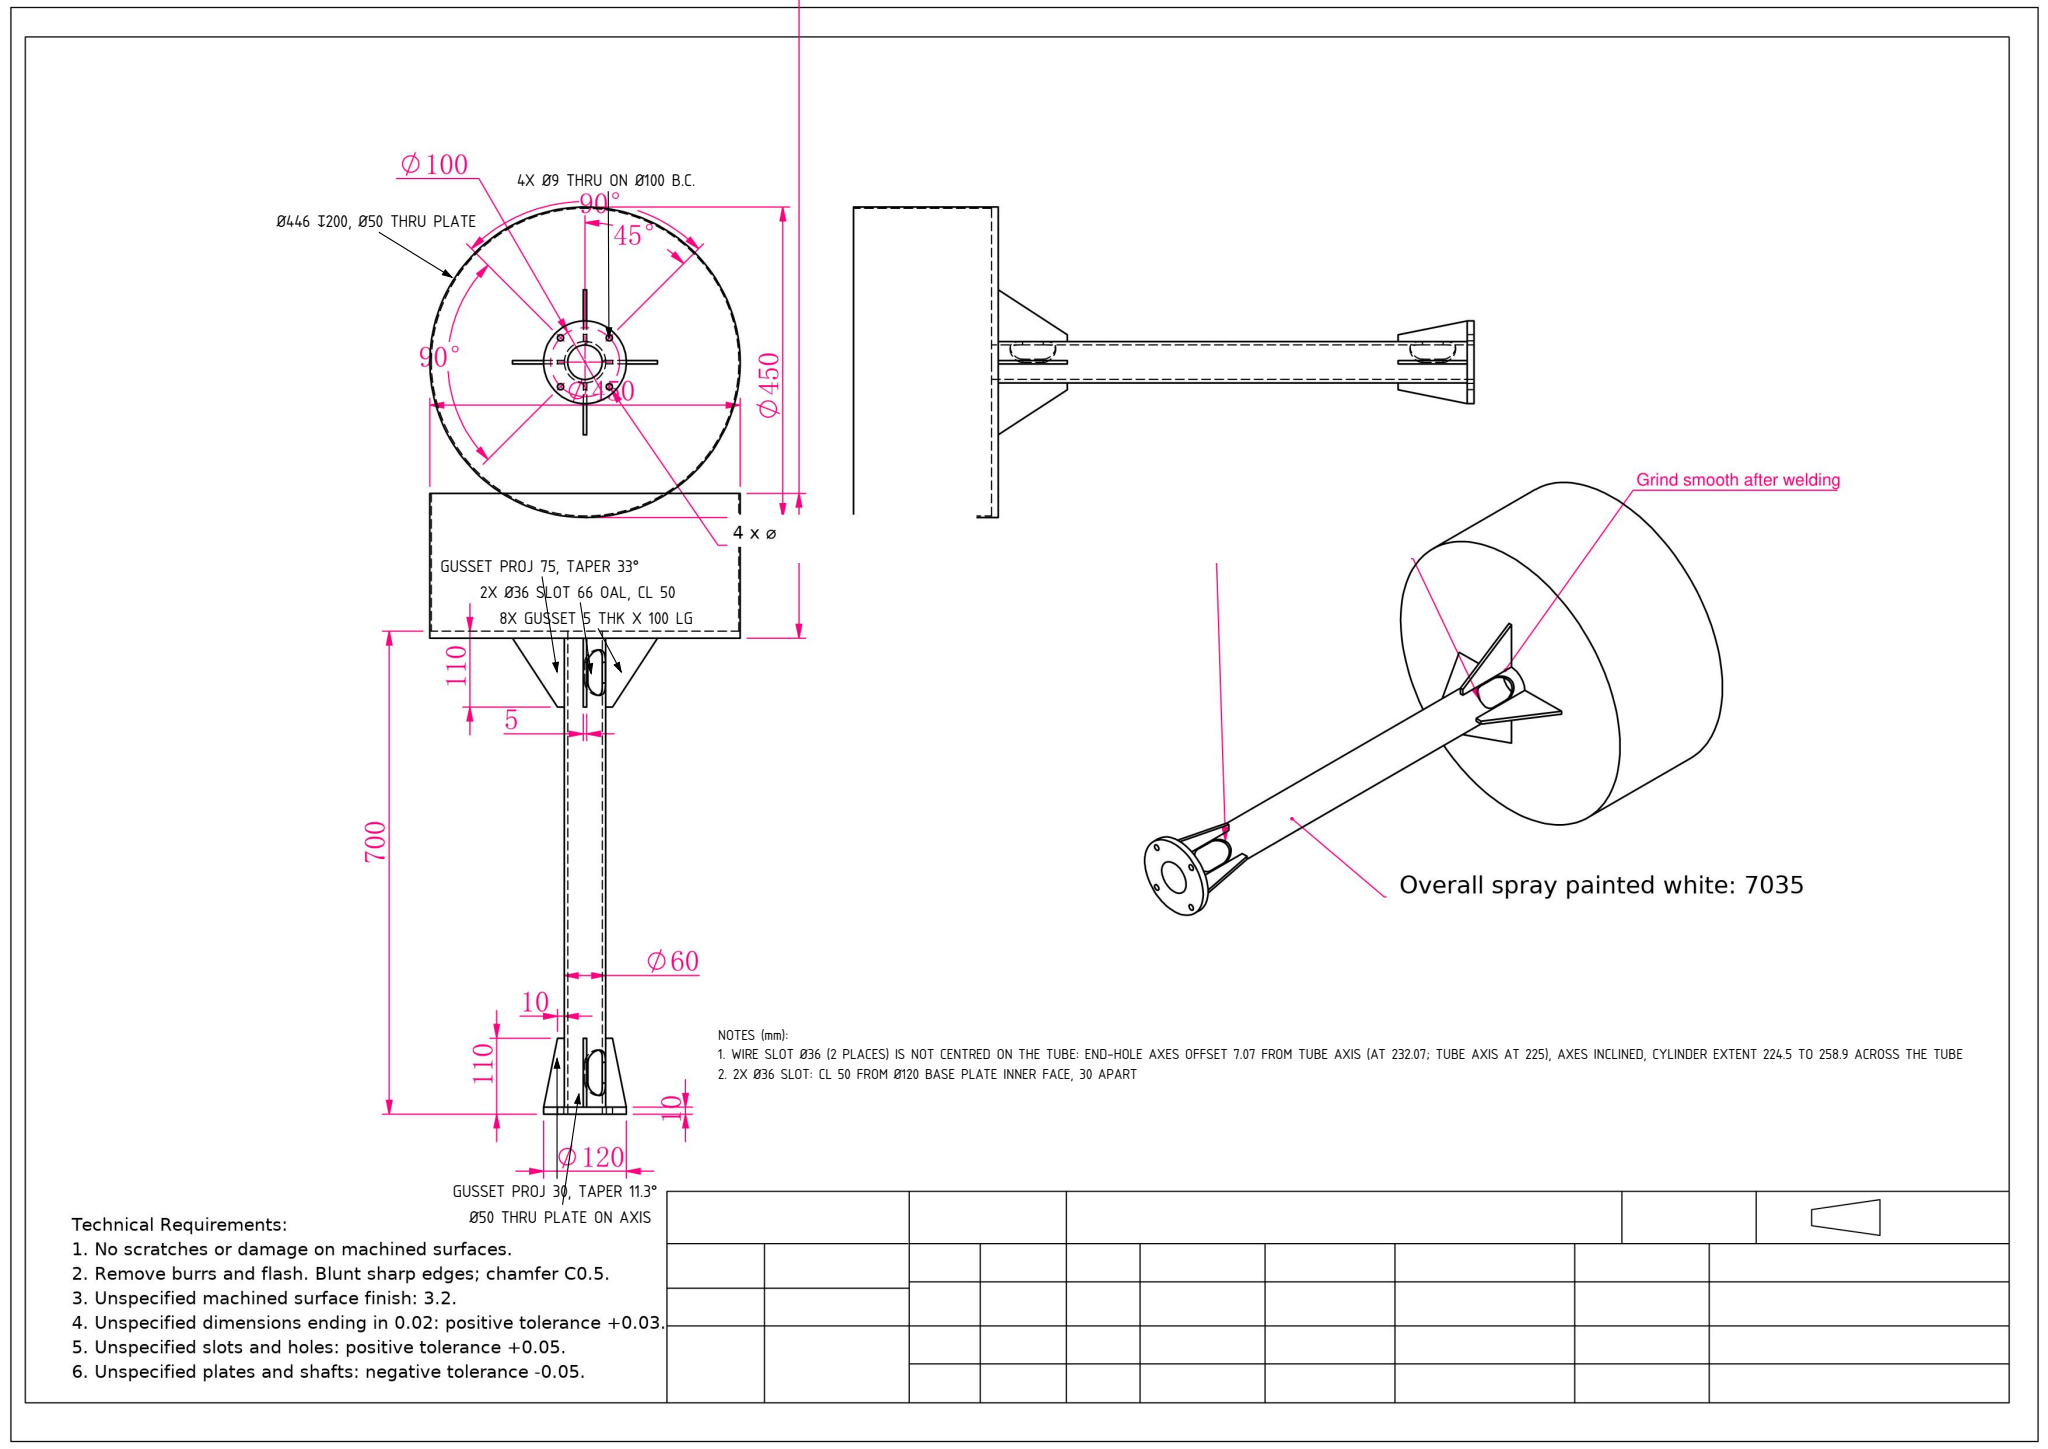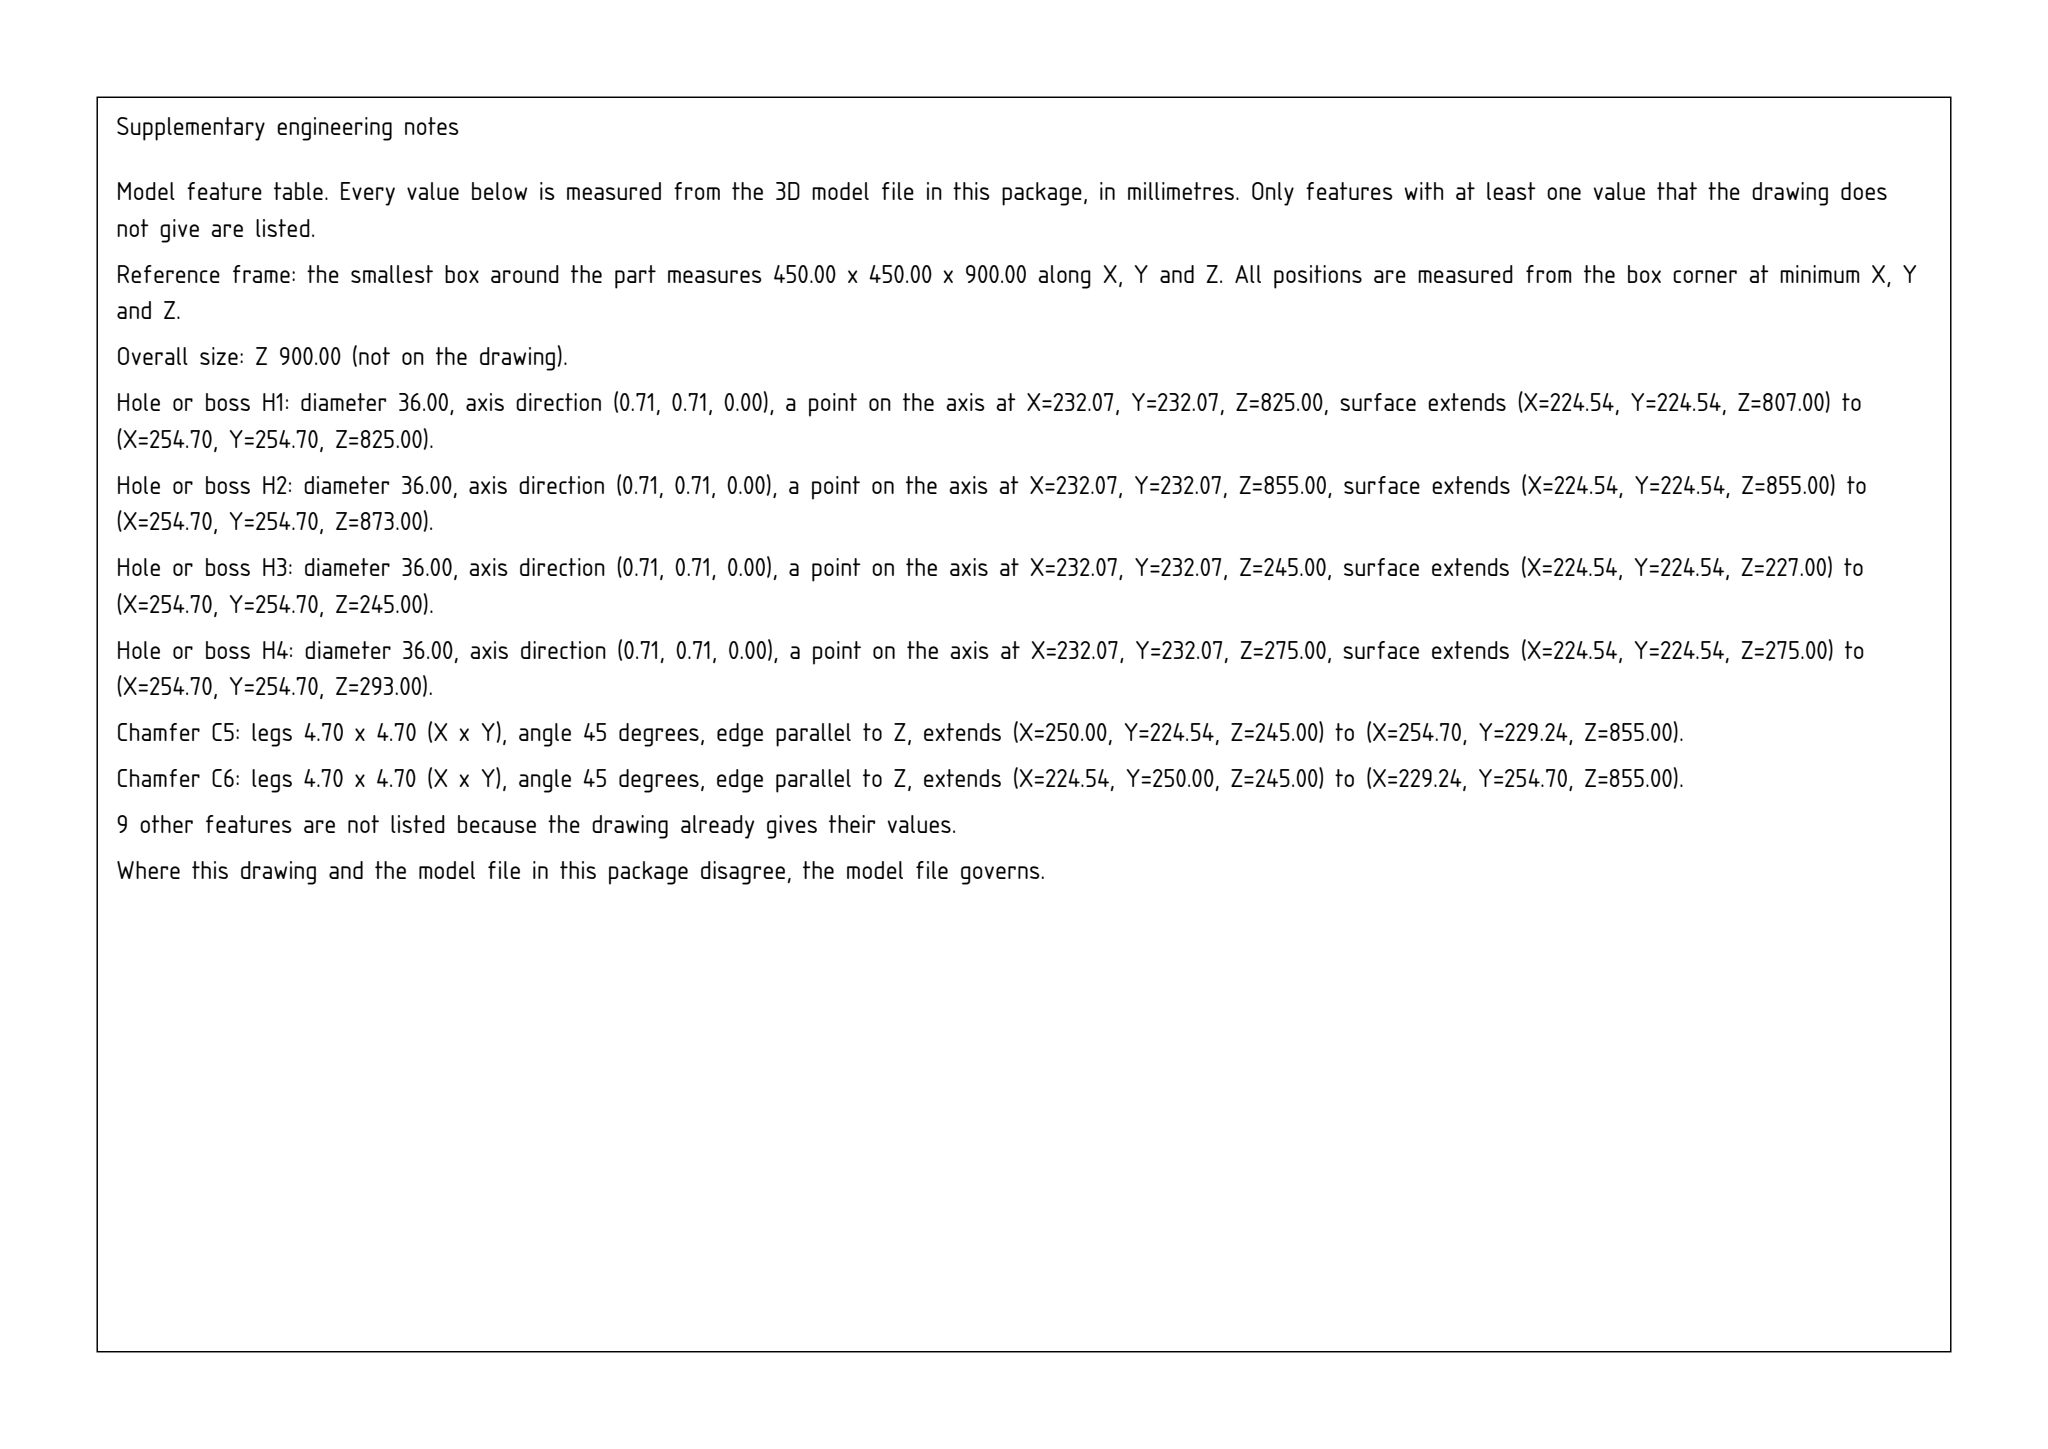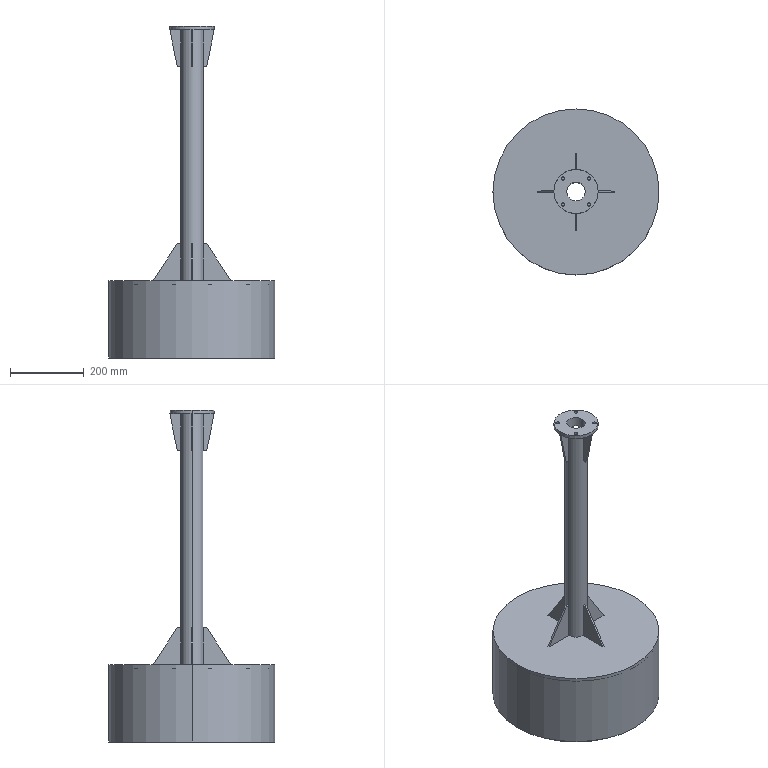Part | SolidWorks | mm | material 45 Steel Chrome Plated | 1 solid | 74 faces | box 450 x 450 x 900 mm | volume 2914669 mm3 | plane 52 | cylinder 22 | commonest cylinder face diameters 9 x8 36 x4 446 x2 450 x2 50 x2 120 x2 60 x2
Drawing notes:
8 GUSSETS 5 THK: FACES AT X=222.5/227.5 AND Y=222.5/227.5 (i.e. 2.5 EACH SIDE OF TUBE AXIS AT 225), 4 EA END AT 90°, RUNNING 100 ALONG TUBE FROM DRUM BACK FACE (Z=210 TO 310) AND FROM BASE PLATE FACE (Z=890 TO 790) | from the solid: axis_planes x=222.5/227.5 (4), y=222.5/227.5 (4), z=310 (4), z=790 (4); tube dia 60 at x=y=225
4 x Ø9 THRU IN BASE PLATE, EQUALLY SPACED ON Ø100 B.C. AT ±35.36 FROM TUBE AXIS IN X AND Y (45° TO GUSSET WEBS); PLATE Ø120 x 10 THK, FACE Z890 TO Z900 | from the solid: cylinders dia 9.0 axis z at (189.64/260.36, 189.64/260.36) L=10; cylinder dia 120 axis z at (225,225) L=10; planes z=890, z=900
WIRE SLOT Ø36 x 66 OAL THRU TUBE, 2 PLACES: END HOLE CENTRES 30 APART (Z245 & Z275, Z825 & Z855); SLOT CL AT Z260 = 50 FROM DRUM BACK FACE (Z210) AND AT Z840 = 50 FROM BASE PLATE FACE (Z890) | from the solid: cylinders dia 36.0 axis x at z=245, 275, 825, 855; planes z=210 and z=890
DRUM-END GUSSETS (4 OFF AT 90°, 5 THK): OUTER EDGE AT R105 FROM TUBE AXIS (X/Y = 120 & 330), i.e. PROJECT 75 FROM Ø60 TUBE OD; 100 LONG ALONG TUBE Z210 TO Z310; TAPERED EDGE 65 x 100 AT 33° TO TUBE AXIS, TIP 10.1 WIDE AT Z310 | from the solid: axis_planes x/y=222.5 & 227.5 extent y/x [120.0,195.1], z [210,310]; inclined_plane angle 33° bbox_from [120,222.5,210] size 65x5x100; z=310 faces 10.1 x 5
BASE-END GUSSETS (4 OFF AT 90°, 5 THK): OUTER EDGE AT R60 FROM TUBE AXIS (X/Y = 165 & 285), i.e. PROJECT 30 FROM Ø60 TUBE OD; 100 LONG ALONG TUBE Z790 TO Z890; TAPERED EDGE 20 x 100 AT 11.3° TO TUBE AXIS, TIP 10.1 WIDE AT Z790 | from the solid: axis_planes x/y=222.5 & 227.5 extent [165.0,195.1] and [254.9,285.0], z [790,890]; inclined_plane angle 11.3° bbox_from [165,222.5,790] size 20x5x100; z=790 faces 10.1 x 5
WIRE SLOT Ø36 (2 PLACES) IS NOT CENTRED ON THE TUBE: END-HOLE AXES OFFSET 7.07 FROM TUBE AXIS (AT 232.07; TUBE AXIS AT 225), AXES INCLINED, CYLINDER EXTENT 224.5 TO 258.9 ACROSS THE TUBE | from the solid: cylinders Ø36 'inclined' axis_pos [232.1, null, 245/275/825/855], from 224.5 to 258.9
DRUM BACK PLATE: Ø446 x 200 DP INTERNAL BORE ENDS AT Z200; Ø50 BORE CONTINUES THRU PLATE Z200-Z210 | from the solid: cylinders: hole/bore Ø446 z from 0 to 200; hole/bore Ø50 z from 200 to 900; boss Ø450 z 0-210
BASE PLATE Ø120 x 10 THK (Z890-Z900): Ø50 BORE THRU PLATE ON TUBE AXIS (225,225) | from the solid: cylinders: boss Ø120 z 890-900; hole/bore Ø50 z 200-900 at (225,225)
2X Ø36 SLOT: CL 50 FROM Ø120 BASE PLATE INNER FACE, 30 APART | from the solid: Ø36 slot arcs at z=825 & 855 (CL 840); base plate z=890-900, inner face z=890 -> 890-840=50; spacing 855-825=30